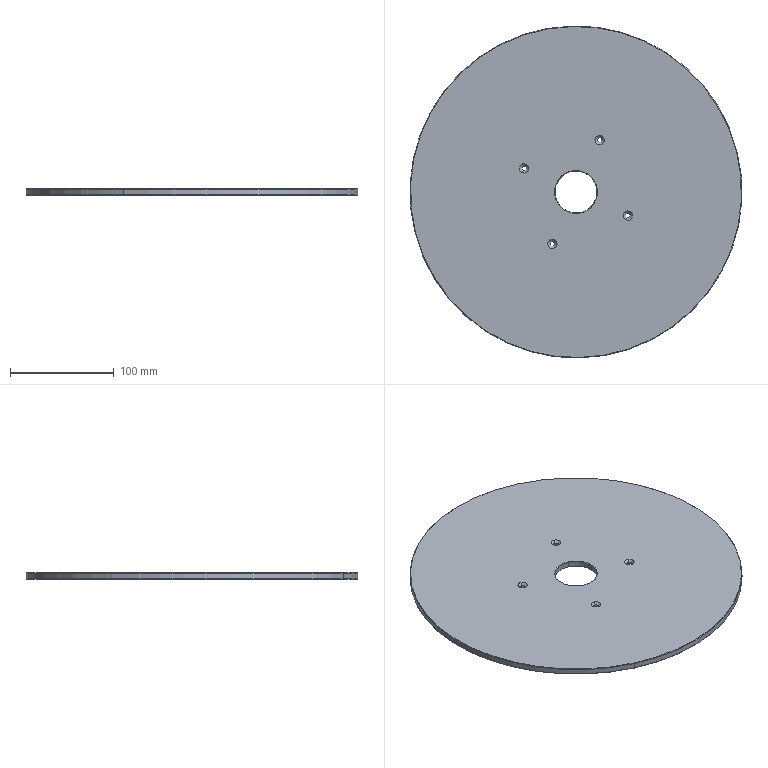Component | SolidWorks | 8TC-A17001-20-04Baffle1-1 | 1 solid | 30 faces | box 320 x 320 x 6 mm | volume 473967 mm3 | cone 16 | cylinder 12 | plane 2 | commonest cylinder face diameters 4.5 x8 40.5 x2 320 x2 | material Tempered Glass
STEP:
#1=COLOUR_RGB('',0.7922,0.8196,0.9333);
#2=FILL_AREA_STYLE_COLOUR('',#1);
#3=FILL_AREA_STYLE('',(#2));
#4=SURFACE_STYLE_FILL_AREA(#3);
#5=SURFACE_SIDE_STYLE('',(#4));
#6=SURFACE_STYLE_USAGE(.BOTH.,#5);
#7=PRESENTATION_STYLE_ASSIGNMENT((#6));
#8=CARTESIAN_POINT('',(26.261,2.186,4.429));
#9=VERTEX_POINT('',#8);
#10=CARTESIAN_POINT('',(31.458,13.619,4.429));
#11=VERTEX_POINT('',#10);
#12=CARTESIAN_POINT('',(28.859,7.902,4.429));
#13=DIRECTION('',(0.,-0.,1.));
#14=DIRECTION('',(-0.4138,-0.9104,0.));
#15=AXIS2_PLACEMENT_3D('',#12,#13,#14);
#16=CIRCLE('',#15,6.28);
#17=EDGE_CURVE('',#9,#11,#16,.T.);
#18=ORIENTED_EDGE('',*,*,#17,.F.);
#19=CARTESIAN_POINT('',(26.253,2.168,4.409));
#20=VERTEX_POINT('',#19);
#21=CARTESIAN_POINT('',(26.261,2.186,4.429));
#22=DIRECTION('',(-0.2926,-0.6437,-0.7071));
#23=VECTOR('',#22,39.37);
#24=LINE('',#21,#23);
#25=EDGE_CURVE('',#9,#20,#24,.T.);
#26=ORIENTED_EDGE('',*,*,#25,.T.);
#27=CARTESIAN_POINT('',(31.466,13.637,4.409));
#28=VERTEX_POINT('',#27);
#29=CARTESIAN_POINT('',(28.859,7.902,4.409));
#30=DIRECTION('',(-0.,0.,-1.));
#31=DIRECTION('',(-0.4138,-0.9104,0.));
#32=AXIS2_PLACEMENT_3D('',#29,#30,#31);
#33=CIRCLE('',#32,6.299);
#34=EDGE_CURVE('',#28,#20,#33,.T.);
#35=ORIENTED_EDGE('',*,*,#34,.F.);
#36=CARTESIAN_POINT('',(31.458,13.619,4.429));
#37=DIRECTION('',(0.2926,0.6437,-0.7071));
#38=VECTOR('',#37,39.37);
#39=LINE('',#36,#38);
#40=EDGE_CURVE('',#11,#28,#39,.T.);
#41=ORIENTED_EDGE('',*,*,#40,.F.);
#42=EDGE_LOOP('',(#18,#26,#35,#41));
#43=FACE_OUTER_BOUND('',#42,.T.);
#44=CARTESIAN_POINT('',(28.859,7.902,4.429));
#45=DIRECTION('',(-0.,0.,-1.));
#46=DIRECTION('',(0.4138,0.9104,0.));
#47=AXIS2_PLACEMENT_3D('',#44,#45,#46);
#48=CONICAL_SURFACE('',#47,6.28,0.7854);
#49=ADVANCED_FACE('',(#43),#48,.T.);
#50=CARTESIAN_POINT('',(31.458,13.619,4.193));
#51=VERTEX_POINT('',#50);
#52=CARTESIAN_POINT('',(26.261,2.186,4.193));
#53=VERTEX_POINT('',#52);
#54=CARTESIAN_POINT('',(28.859,7.902,4.193));
#55=DIRECTION('',(-0.,0.,-1.));
#56=DIRECTION('',(-0.4138,-0.9104,0.));
#57=AXIS2_PLACEMENT_3D('',#54,#55,#56);
#58=CIRCLE('',#57,6.28);
#59=EDGE_CURVE('',#51,#53,#58,.T.);
#60=ORIENTED_EDGE('',*,*,#59,.F.);
#61=CARTESIAN_POINT('',(31.466,13.637,4.213));
#62=VERTEX_POINT('',#61);
#63=CARTESIAN_POINT('',(31.466,13.637,4.213));
#64=DIRECTION('',(0.2926,0.6437,0.7071));
#65=VECTOR('',#64,39.37);
#66=LINE('',#63,#65);
#67=EDGE_CURVE('',#51,#62,#66,.T.);
#68=ORIENTED_EDGE('',*,*,#67,.T.);
#69=CARTESIAN_POINT('',(26.253,2.168,4.213));
#70=VERTEX_POINT('',#69);
#71=CARTESIAN_POINT('',(28.859,7.902,4.213));
#72=DIRECTION('',(0.,-0.,1.));
#73=DIRECTION('',(-0.4138,-0.9104,0.));
#74=AXIS2_PLACEMENT_3D('',#71,#72,#73);
#75=CIRCLE('',#74,6.299);
#76=EDGE_CURVE('',#70,#62,#75,.T.);
#77=ORIENTED_EDGE('',*,*,#76,.F.);
#78=CARTESIAN_POINT('',(26.253,2.168,4.213));
#79=DIRECTION('',(-0.2926,-0.6437,0.7071));
#80=VECTOR('',#79,39.37);
#81=LINE('',#78,#80);
#82=EDGE_CURVE('',#53,#70,#81,.T.);
#83=ORIENTED_EDGE('',*,*,#82,.F.);
#84=EDGE_LOOP('',(#60,#68,#77,#83));
#85=FACE_OUTER_BOUND('',#84,.T.);
#86=CARTESIAN_POINT('',(28.859,7.902,4.213));
#87=DIRECTION('',(0.,-0.,1.));
#88=DIRECTION('',(-0.4138,-0.9104,0.));
#89=AXIS2_PLACEMENT_3D('',#86,#87,#88);
#90=CONICAL_SURFACE('',#89,6.299,0.7854);
#91=ADVANCED_FACE('',(#85),#90,.T.);
#92=CARTESIAN_POINT('',(29.189,8.628,4.409));
#93=VERTEX_POINT('',#92);
#94=CARTESIAN_POINT('',(28.53,7.177,4.409));
#95=VERTEX_POINT('',#94);
#96=CARTESIAN_POINT('',(28.859,7.902,4.409));
#97=DIRECTION('',(0.,-0.,1.));
#98=DIRECTION('',(-0.4138,-0.9104,0.));
#99=AXIS2_PLACEMENT_3D('',#96,#97,#98);
#100=CIRCLE('',#99,0.7972);
#101=EDGE_CURVE('',#93,#95,#100,.T.);
#102=ORIENTED_EDGE('',*,*,#101,.F.);
#103=CARTESIAN_POINT('',(29.197,8.646,4.429));
#104=VERTEX_POINT('',#103);
#105=CARTESIAN_POINT('',(29.189,8.628,4.409));
#106=DIRECTION('',(0.2926,0.6437,0.7071));
#107=VECTOR('',#106,39.37);
#108=LINE('',#105,#107);
#109=EDGE_CURVE('',#93,#104,#108,.T.);
#110=ORIENTED_EDGE('',*,*,#109,.T.);
#111=CARTESIAN_POINT('',(28.521,7.159,4.429));
#112=VERTEX_POINT('',#111);
#113=CARTESIAN_POINT('',(28.859,7.902,4.429));
#114=DIRECTION('',(-0.,0.,-1.));
#115=DIRECTION('',(-0.4138,-0.9104,0.));
#116=AXIS2_PLACEMENT_3D('',#113,#114,#115);
#117=CIRCLE('',#116,0.8169);
#118=EDGE_CURVE('',#112,#104,#117,.T.);
#119=ORIENTED_EDGE('',*,*,#118,.F.);
#120=CARTESIAN_POINT('',(28.53,7.177,4.409));
#121=DIRECTION('',(-0.2926,-0.6437,0.7071));
#122=VECTOR('',#121,39.37);
#123=LINE('',#120,#122);
#124=EDGE_CURVE('',#95,#112,#123,.T.);
#125=ORIENTED_EDGE('',*,*,#124,.F.);
#126=EDGE_LOOP('',(#102,#110,#119,#125));
#127=FACE_OUTER_BOUND('',#126,.T.);
#128=CARTESIAN_POINT('',(28.859,7.902,4.409));
#129=DIRECTION('',(0.,-0.,1.));
#130=DIRECTION('',(-0.4138,-0.9104,0.));
#131=AXIS2_PLACEMENT_3D('',#128,#129,#130);
#132=CONICAL_SURFACE('',#131,0.7972,0.7854);
#133=ADVANCED_FACE('',(#127),#132,.F.);
#134=CARTESIAN_POINT('',(28.53,7.177,4.213));
#135=VERTEX_POINT('',#134);
#136=CARTESIAN_POINT('',(29.189,8.628,4.213));
#137=VERTEX_POINT('',#136);
#138=CARTESIAN_POINT('',(28.859,7.902,4.213));
#139=DIRECTION('',(-0.,0.,-1.));
#140=DIRECTION('',(-0.4138,-0.9104,0.));
#141=AXIS2_PLACEMENT_3D('',#138,#139,#140);
#142=CIRCLE('',#141,0.7972);
#143=EDGE_CURVE('',#135,#137,#142,.T.);
#144=ORIENTED_EDGE('',*,*,#143,.F.);
#145=CARTESIAN_POINT('',(28.521,7.159,4.193));
#146=VERTEX_POINT('',#145);
#147=CARTESIAN_POINT('',(28.521,7.159,4.193));
#148=DIRECTION('',(-0.2926,-0.6437,-0.7071));
#149=VECTOR('',#148,39.37);
#150=LINE('',#147,#149);
#151=EDGE_CURVE('',#135,#146,#150,.T.);
#152=ORIENTED_EDGE('',*,*,#151,.T.);
#153=CARTESIAN_POINT('',(29.197,8.646,4.193));
#154=VERTEX_POINT('',#153);
#155=CARTESIAN_POINT('',(28.859,7.902,4.193));
#156=DIRECTION('',(0.,-0.,1.));
#157=DIRECTION('',(-0.4138,-0.9104,0.));
#158=AXIS2_PLACEMENT_3D('',#155,#156,#157);
#159=CIRCLE('',#158,0.8169);
#160=EDGE_CURVE('',#154,#146,#159,.T.);
#161=ORIENTED_EDGE('',*,*,#160,.F.);
#162=CARTESIAN_POINT('',(29.197,8.646,4.193));
#163=DIRECTION('',(0.2926,0.6437,-0.7071));
#164=VECTOR('',#163,39.37);
#165=LINE('',#162,#164);
#166=EDGE_CURVE('',#137,#154,#165,.T.);
#167=ORIENTED_EDGE('',*,*,#166,.F.);
#168=EDGE_LOOP('',(#144,#152,#161,#167));
#169=FACE_OUTER_BOUND('',#168,.T.);
#170=CARTESIAN_POINT('',(28.859,7.902,4.193));
#171=DIRECTION('',(-0.,0.,-1.));
#172=DIRECTION('',(0.4138,0.9104,0.));
#173=AXIS2_PLACEMENT_3D('',#170,#171,#172);
#174=CONICAL_SURFACE('',#173,0.8169,0.7854);
#175=ADVANCED_FACE('',(#169),#174,.F.);
#176=CARTESIAN_POINT('',(30.867,7.087,4.341));
#177=VERTEX_POINT('',#176);
#178=CARTESIAN_POINT('',(30.794,6.926,4.341));
#179=VERTEX_POINT('',#178);
#180=CARTESIAN_POINT('',(30.831,7.006,4.341));
#181=DIRECTION('',(0.,-0.,1.));
#182=DIRECTION('',(-0.4138,-0.9104,0.));
#183=AXIS2_PLACEMENT_3D('',#180,#181,#182);
#184=CIRCLE('',#183,0.08858);
#185=EDGE_CURVE('',#177,#179,#184,.T.);
#186=ORIENTED_EDGE('',*,*,#185,.F.);
#187=CARTESIAN_POINT('',(30.904,7.167,4.429));
#188=VERTEX_POINT('',#187);
#189=CARTESIAN_POINT('',(30.904,7.167,4.429));
#190=DIRECTION('',(0.2926,0.6437,0.7071));
#191=VECTOR('',#190,39.37);
#192=LINE('',#189,#191);
#193=EDGE_CURVE('',#177,#188,#192,.T.);
#194=ORIENTED_EDGE('',*,*,#193,.T.);
#195=CARTESIAN_POINT('',(30.758,6.846,4.429));
#196=VERTEX_POINT('',#195);
#197=CARTESIAN_POINT('',(30.831,7.006,4.429));
#198=DIRECTION('',(0.,-0.,1.));
#199=DIRECTION('',(-0.4138,-0.9104,0.));
#200=AXIS2_PLACEMENT_3D('',#197,#198,#199);
#201=CIRCLE('',#200,0.1764);
#202=EDGE_CURVE('',#188,#196,#201,.T.);
#203=ORIENTED_EDGE('',*,*,#202,.T.);
#204=CARTESIAN_POINT('',(30.758,6.846,4.429));
#205=DIRECTION('',(-0.2926,-0.6437,0.7071));
#206=VECTOR('',#205,39.37);
#207=LINE('',#204,#206);
#208=EDGE_CURVE('',#179,#196,#207,.T.);
#209=ORIENTED_EDGE('',*,*,#208,.F.);
#210=EDGE_LOOP('',(#186,#194,#203,#209));
#211=FACE_OUTER_BOUND('',#210,.T.);
#212=CARTESIAN_POINT('',(30.831,7.006,4.429));
#213=DIRECTION('',(0.,-0.,1.));
#214=DIRECTION('',(-0.4138,-0.9104,0.));
#215=AXIS2_PLACEMENT_3D('',#212,#213,#214);
#216=CONICAL_SURFACE('',#215,0.1764,0.7854);
#217=ADVANCED_FACE('',(#211),#216,.F.);
#218=CARTESIAN_POINT('',(30.867,7.087,4.193));
#219=VERTEX_POINT('',#218);
#220=CARTESIAN_POINT('',(30.794,6.926,4.193));
#221=VERTEX_POINT('',#220);
#222=CARTESIAN_POINT('',(30.831,7.006,4.193));
#223=DIRECTION('',(0.,-0.,1.));
#224=DIRECTION('',(-0.4138,-0.9104,0.));
#225=AXIS2_PLACEMENT_3D('',#222,#223,#224);
#226=CIRCLE('',#225,0.08858);
#227=EDGE_CURVE('',#219,#221,#226,.T.);
#228=ORIENTED_EDGE('',*,*,#227,.F.);
#229=CARTESIAN_POINT('',(30.867,7.087,4.429));
#230=DIRECTION('',(0.,-0.,1.));
#231=VECTOR('',#230,39.37);
#232=LINE('',#229,#231);
#233=EDGE_CURVE('',#219,#177,#232,.T.);
#234=ORIENTED_EDGE('',*,*,#233,.T.);
#235=ORIENTED_EDGE('',*,*,#185,.T.);
#236=CARTESIAN_POINT('',(30.794,6.926,4.429));
#237=DIRECTION('',(0.,-0.,1.));
#238=VECTOR('',#237,39.37);
#239=LINE('',#236,#238);
#240=EDGE_CURVE('',#221,#179,#239,.T.);
#241=ORIENTED_EDGE('',*,*,#240,.F.);
#242=EDGE_LOOP('',(#228,#234,#235,#241));
#243=FACE_OUTER_BOUND('',#242,.T.);
#244=CARTESIAN_POINT('',(30.831,7.006,4.429));
#245=DIRECTION('',(0.,-0.,1.));
#246=DIRECTION('',(-0.4138,-0.9104,0.));
#247=AXIS2_PLACEMENT_3D('',#244,#245,#246);
#248=CYLINDRICAL_SURFACE('',#247,0.08858);
#249=ADVANCED_FACE('',(#243),#248,.F.);
#250=CARTESIAN_POINT('',(29.792,9.954,4.341));
#251=VERTEX_POINT('',#250);
#252=CARTESIAN_POINT('',(29.719,9.793,4.341));
#253=VERTEX_POINT('',#252);
#254=CARTESIAN_POINT('',(29.755,9.874,4.341));
#255=DIRECTION('',(0.,-0.,1.));
#256=DIRECTION('',(-0.4138,-0.9104,0.));
#257=AXIS2_PLACEMENT_3D('',#254,#255,#256);
#258=CIRCLE('',#257,0.08858);
#259=EDGE_CURVE('',#251,#253,#258,.T.);
#260=ORIENTED_EDGE('',*,*,#259,.F.);
#261=CARTESIAN_POINT('',(29.828,10.034,4.429));
#262=VERTEX_POINT('',#261);
#263=CARTESIAN_POINT('',(29.828,10.034,4.429));
#264=DIRECTION('',(0.2926,0.6437,0.7071));
#265=VECTOR('',#264,39.37);
#266=LINE('',#263,#265);
#267=EDGE_CURVE('',#251,#262,#266,.T.);
#268=ORIENTED_EDGE('',*,*,#267,.T.);
#269=CARTESIAN_POINT('',(29.682,9.713,4.429));
#270=VERTEX_POINT('',#269);
#271=CARTESIAN_POINT('',(29.755,9.874,4.429));
#272=DIRECTION('',(0.,-0.,1.));
#273=DIRECTION('',(-0.4138,-0.9104,0.));
#274=AXIS2_PLACEMENT_3D('',#271,#272,#273);
#275=CIRCLE('',#274,0.1764);
#276=EDGE_CURVE('',#262,#270,#275,.T.);
#277=ORIENTED_EDGE('',*,*,#276,.T.);
#278=CARTESIAN_POINT('',(29.682,9.713,4.429));
#279=DIRECTION('',(-0.2926,-0.6437,0.7071));
#280=VECTOR('',#279,39.37);
#281=LINE('',#278,#280);
#282=EDGE_CURVE('',#253,#270,#281,.T.);
#283=ORIENTED_EDGE('',*,*,#282,.F.);
#284=EDGE_LOOP('',(#260,#268,#277,#283));
#285=FACE_OUTER_BOUND('',#284,.T.);
#286=CARTESIAN_POINT('',(29.755,9.874,4.429));
#287=DIRECTION('',(0.,-0.,1.));
#288=DIRECTION('',(-0.4138,-0.9104,0.));
#289=AXIS2_PLACEMENT_3D('',#286,#287,#288);
#290=CONICAL_SURFACE('',#289,0.1764,0.7854);
#291=ADVANCED_FACE('',(#285),#290,.F.);
#292=CARTESIAN_POINT('',(29.792,9.954,4.193));
#293=VERTEX_POINT('',#292);
#294=CARTESIAN_POINT('',(29.719,9.793,4.193));
#295=VERTEX_POINT('',#294);
#296=CARTESIAN_POINT('',(29.755,9.874,4.193));
#297=DIRECTION('',(0.,-0.,1.));
#298=DIRECTION('',(-0.4138,-0.9104,0.));
#299=AXIS2_PLACEMENT_3D('',#296,#297,#298);
#300=CIRCLE('',#299,0.08858);
#301=EDGE_CURVE('',#293,#295,#300,.T.);
#302=ORIENTED_EDGE('',*,*,#301,.F.);
#303=CARTESIAN_POINT('',(29.792,9.954,4.429));
#304=DIRECTION('',(0.,-0.,1.));
#305=VECTOR('',#304,39.37);
#306=LINE('',#303,#305);
#307=EDGE_CURVE('',#293,#251,#306,.T.);
#308=ORIENTED_EDGE('',*,*,#307,.T.);
#309=ORIENTED_EDGE('',*,*,#259,.T.);
#310=CARTESIAN_POINT('',(29.719,9.793,4.429));
#311=DIRECTION('',(0.,-0.,1.));
#312=VECTOR('',#311,39.37);
#313=LINE('',#310,#312);
#314=EDGE_CURVE('',#295,#253,#313,.T.);
#315=ORIENTED_EDGE('',*,*,#314,.F.);
#316=EDGE_LOOP('',(#302,#308,#309,#315));
#317=FACE_OUTER_BOUND('',#316,.T.);
#318=CARTESIAN_POINT('',(29.755,9.874,4.429));
#319=DIRECTION('',(0.,-0.,1.));
#320=DIRECTION('',(-0.4138,-0.9104,0.));
#321=AXIS2_PLACEMENT_3D('',#318,#319,#320);
#322=CYLINDRICAL_SURFACE('',#321,0.08858);
#323=ADVANCED_FACE('',(#317),#322,.F.);
#324=CARTESIAN_POINT('',(28.,6.012,4.341));
#325=VERTEX_POINT('',#324);
#326=CARTESIAN_POINT('',(27.927,5.851,4.341));
#327=VERTEX_POINT('',#326);
#328=CARTESIAN_POINT('',(27.963,5.931,4.341));
#329=DIRECTION('',(0.,-0.,1.));
#330=DIRECTION('',(-0.4138,-0.9104,0.));
#331=AXIS2_PLACEMENT_3D('',#328,#329,#330);
#332=CIRCLE('',#331,0.08858);
#333=EDGE_CURVE('',#325,#327,#332,.T.);
#334=ORIENTED_EDGE('',*,*,#333,.F.);
#335=CARTESIAN_POINT('',(28.036,6.092,4.429));
#336=VERTEX_POINT('',#335);
#337=CARTESIAN_POINT('',(28.036,6.092,4.429));
#338=DIRECTION('',(0.2926,0.6437,0.7071));
#339=VECTOR('',#338,39.37);
#340=LINE('',#337,#339);
#341=EDGE_CURVE('',#325,#336,#340,.T.);
#342=ORIENTED_EDGE('',*,*,#341,.T.);
#343=CARTESIAN_POINT('',(27.89,5.771,4.429));
#344=VERTEX_POINT('',#343);
#345=CARTESIAN_POINT('',(27.963,5.931,4.429));
#346=DIRECTION('',(0.,-0.,1.));
#347=DIRECTION('',(-0.4138,-0.9104,0.));
#348=AXIS2_PLACEMENT_3D('',#345,#346,#347);
#349=CIRCLE('',#348,0.1764);
#350=EDGE_CURVE('',#336,#344,#349,.T.);
#351=ORIENTED_EDGE('',*,*,#350,.T.);
#352=CARTESIAN_POINT('',(27.89,5.771,4.429));
#353=DIRECTION('',(-0.2926,-0.6437,0.7071));
#354=VECTOR('',#353,39.37);
#355=LINE('',#352,#354);
#356=EDGE_CURVE('',#327,#344,#355,.T.);
#357=ORIENTED_EDGE('',*,*,#356,.F.);
#358=EDGE_LOOP('',(#334,#342,#351,#357));
#359=FACE_OUTER_BOUND('',#358,.T.);
#360=CARTESIAN_POINT('',(27.963,5.931,4.429));
#361=DIRECTION('',(0.,-0.,1.));
#362=DIRECTION('',(-0.4138,-0.9104,0.));
#363=AXIS2_PLACEMENT_3D('',#360,#361,#362);
#364=CONICAL_SURFACE('',#363,0.1764,0.7854);
#365=ADVANCED_FACE('',(#359),#364,.F.);
#366=CARTESIAN_POINT('',(28.,6.012,4.193));
#367=VERTEX_POINT('',#366);
#368=CARTESIAN_POINT('',(27.927,5.851,4.193));
#369=VERTEX_POINT('',#368);
#370=CARTESIAN_POINT('',(27.963,5.931,4.193));
#371=DIRECTION('',(0.,-0.,1.));
#372=DIRECTION('',(-0.4138,-0.9104,0.));
#373=AXIS2_PLACEMENT_3D('',#370,#371,#372);
#374=CIRCLE('',#373,0.08858);
#375=EDGE_CURVE('',#367,#369,#374,.T.);
#376=ORIENTED_EDGE('',*,*,#375,.F.);
#377=CARTESIAN_POINT('',(28.,6.012,4.429));
#378=DIRECTION('',(0.,-0.,1.));
#379=VECTOR('',#378,39.37);
#380=LINE('',#377,#379);
#381=EDGE_CURVE('',#367,#325,#380,.T.);
#382=ORIENTED_EDGE('',*,*,#381,.T.);
#383=ORIENTED_EDGE('',*,*,#333,.T.);
#384=CARTESIAN_POINT('',(27.927,5.851,4.429));
#385=DIRECTION('',(0.,-0.,1.));
#386=VECTOR('',#385,39.37);
#387=LINE('',#384,#386);
#388=EDGE_CURVE('',#369,#327,#387,.T.);
#389=ORIENTED_EDGE('',*,*,#388,.F.);
#390=EDGE_LOOP('',(#376,#382,#383,#389));
#391=FACE_OUTER_BOUND('',#390,.T.);
#392=CARTESIAN_POINT('',(27.963,5.931,4.429));
#393=DIRECTION('',(0.,-0.,1.));
#394=DIRECTION('',(-0.4138,-0.9104,0.));
#395=AXIS2_PLACEMENT_3D('',#392,#393,#394);
#396=CYLINDRICAL_SURFACE('',#395,0.08858);
#397=ADVANCED_FACE('',(#391),#396,.F.);
#398=CARTESIAN_POINT('',(26.925,8.879,4.341));
#399=VERTEX_POINT('',#398);
#400=CARTESIAN_POINT('',(26.851,8.718,4.341));
#401=VERTEX_POINT('',#400);
#402=CARTESIAN_POINT('',(26.888,8.798,4.341));
#403=DIRECTION('',(0.,-0.,1.));
#404=DIRECTION('',(-0.4138,-0.9104,0.));
#405=AXIS2_PLACEMENT_3D('',#402,#403,#404);
#406=CIRCLE('',#405,0.08858);
#407=EDGE_CURVE('',#399,#401,#406,.T.);
#408=ORIENTED_EDGE('',*,*,#407,.F.);
#409=CARTESIAN_POINT('',(26.961,8.959,4.429));
#410=VERTEX_POINT('',#409);
#411=CARTESIAN_POINT('',(26.961,8.959,4.429));
#412=DIRECTION('',(0.2926,0.6437,0.7071));
#413=VECTOR('',#412,39.37);
#414=LINE('',#411,#413);
#415=EDGE_CURVE('',#399,#410,#414,.T.);
#416=ORIENTED_EDGE('',*,*,#415,.T.);
#417=CARTESIAN_POINT('',(26.815,8.638,4.429));
#418=VERTEX_POINT('',#417);
#419=CARTESIAN_POINT('',(26.888,8.798,4.429));
#420=DIRECTION('',(0.,-0.,1.));
#421=DIRECTION('',(-0.4138,-0.9104,0.));
#422=AXIS2_PLACEMENT_3D('',#419,#420,#421);
#423=CIRCLE('',#422,0.1764);
#424=EDGE_CURVE('',#410,#418,#423,.T.);
#425=ORIENTED_EDGE('',*,*,#424,.T.);
#426=CARTESIAN_POINT('',(26.815,8.638,4.429));
#427=DIRECTION('',(-0.2926,-0.6437,0.7071));
#428=VECTOR('',#427,39.37);
#429=LINE('',#426,#428);
#430=EDGE_CURVE('',#401,#418,#429,.T.);
#431=ORIENTED_EDGE('',*,*,#430,.F.);
#432=EDGE_LOOP('',(#408,#416,#425,#431));
#433=FACE_OUTER_BOUND('',#432,.T.);
#434=CARTESIAN_POINT('',(26.888,8.798,4.429));
#435=DIRECTION('',(0.,-0.,1.));
#436=DIRECTION('',(-0.4138,-0.9104,0.));
#437=AXIS2_PLACEMENT_3D('',#434,#435,#436);
#438=CONICAL_SURFACE('',#437,0.1764,0.7854);
#439=ADVANCED_FACE('',(#433),#438,.F.);
#440=CARTESIAN_POINT('',(26.925,8.879,4.193));
#441=VERTEX_POINT('',#440);
#442=CARTESIAN_POINT('',(26.851,8.718,4.193));
#443=VERTEX_POINT('',#442);
#444=CARTESIAN_POINT('',(26.888,8.798,4.193));
#445=DIRECTION('',(0.,-0.,1.));
#446=DIRECTION('',(-0.4138,-0.9104,0.));
#447=AXIS2_PLACEMENT_3D('',#444,#445,#446);
#448=CIRCLE('',#447,0.08858);
#449=EDGE_CURVE('',#441,#443,#448,.T.);
#450=ORIENTED_EDGE('',*,*,#449,.F.);
#451=CARTESIAN_POINT('',(26.925,8.879,4.429));
#452=DIRECTION('',(0.,-0.,1.));
#453=VECTOR('',#452,39.37);
#454=LINE('',#451,#453);
#455=EDGE_CURVE('',#441,#399,#454,.T.);
#456=ORIENTED_EDGE('',*,*,#455,.T.);
#457=ORIENTED_EDGE('',*,*,#407,.T.);
#458=CARTESIAN_POINT('',(26.851,8.718,4.429));
#459=DIRECTION('',(0.,-0.,1.));
#460=VECTOR('',#459,39.37);
#461=LINE('',#458,#460);
#462=EDGE_CURVE('',#443,#401,#461,.T.);
#463=ORIENTED_EDGE('',*,*,#462,.F.);
#464=EDGE_LOOP('',(#450,#456,#457,#463));
#465=FACE_OUTER_BOUND('',#464,.T.);
#466=CARTESIAN_POINT('',(26.888,8.798,4.429));
#467=DIRECTION('',(0.,-0.,1.));
#468=DIRECTION('',(-0.4138,-0.9104,0.));
#469=AXIS2_PLACEMENT_3D('',#466,#467,#468);
#470=CYLINDRICAL_SURFACE('',#469,0.08858);
#471=ADVANCED_FACE('',(#465),#470,.F.);
#472=ORIENTED_EDGE('',*,*,#101,.T.);
#473=CARTESIAN_POINT('',(28.53,7.177,4.429));
#474=DIRECTION('',(-0.,0.,-1.));
#475=VECTOR('',#474,39.37);
#476=LINE('',#473,#475);
#477=EDGE_CURVE('',#95,#135,#476,.T.);
#478=ORIENTED_EDGE('',*,*,#477,.T.);
#479=ORIENTED_EDGE('',*,*,#143,.T.);
#480=CARTESIAN_POINT('',(29.189,8.628,4.429));
#481=DIRECTION('',(-0.,0.,-1.));
#482=VECTOR('',#481,39.37);
#483=LINE('',#480,#482);
#484=EDGE_CURVE('',#93,#137,#483,.T.);
#485=ORIENTED_EDGE('',*,*,#484,.F.);
#486=EDGE_LOOP('',(#472,#478,#479,#485));
#487=FACE_OUTER_BOUND('',#486,.T.);
#488=CARTESIAN_POINT('',(28.859,7.902,4.429));
#489=DIRECTION('',(-0.,0.,-1.));
#490=DIRECTION('',(0.4138,0.9104,0.));
#491=AXIS2_PLACEMENT_3D('',#488,#489,#490);
#492=CYLINDRICAL_SURFACE('',#491,0.7972);
#493=ADVANCED_FACE('',(#487),#492,.F.);
#494=ORIENTED_EDGE('',*,*,#34,.T.);
#495=CARTESIAN_POINT('',(26.253,2.168,4.429));
#496=DIRECTION('',(-0.,0.,-1.));
#497=VECTOR('',#496,39.37);
#498=LINE('',#495,#497);
#499=EDGE_CURVE('',#20,#70,#498,.T.);
#500=ORIENTED_EDGE('',*,*,#499,.T.);
#501=ORIENTED_EDGE('',*,*,#76,.T.);
#502=CARTESIAN_POINT('',(31.466,13.637,4.429));
#503=DIRECTION('',(-0.,0.,-1.));
#504=VECTOR('',#503,39.37);
#505=LINE('',#502,#504);
#506=EDGE_CURVE('',#28,#62,#505,.T.);
#507=ORIENTED_EDGE('',*,*,#506,.F.);
#508=EDGE_LOOP('',(#494,#500,#501,#507));
#509=FACE_OUTER_BOUND('',#508,.T.);
#510=CARTESIAN_POINT('',(28.859,7.902,4.429));
#511=DIRECTION('',(-0.,0.,-1.));
#512=DIRECTION('',(0.4138,0.9104,0.));
#513=AXIS2_PLACEMENT_3D('',#510,#511,#512);
#514=CYLINDRICAL_SURFACE('',#513,6.299);
#515=ADVANCED_FACE('',(#509),#514,.T.);
#516=ORIENTED_EDGE('',*,*,#118,.T.);
#517=CARTESIAN_POINT('',(28.859,7.902,4.429));
#518=DIRECTION('',(-0.,0.,-1.));
#519=DIRECTION('',(-0.4138,-0.9104,0.));
#520=AXIS2_PLACEMENT_3D('',#517,#518,#519);
#521=CIRCLE('',#520,0.8169);
#522=EDGE_CURVE('',#104,#112,#521,.T.);
#523=ORIENTED_EDGE('',*,*,#522,.T.);
#524=EDGE_LOOP('',(#516,#523));
#525=FACE_BOUND('',#524,.T.);
#526=CARTESIAN_POINT('',(28.859,7.902,4.429));
#527=DIRECTION('',(0.,-0.,1.));
#528=DIRECTION('',(-0.4138,-0.9104,0.));
#529=AXIS2_PLACEMENT_3D('',#526,#527,#528);
#530=CIRCLE('',#529,6.28);
#531=EDGE_CURVE('',#11,#9,#530,.T.);
#532=ORIENTED_EDGE('',*,*,#531,.T.);
#533=ORIENTED_EDGE('',*,*,#17,.T.);
#534=EDGE_LOOP('',(#532,#533));
#535=FACE_OUTER_BOUND('',#534,.T.);
#536=CARTESIAN_POINT('',(30.831,7.006,4.429));
#537=DIRECTION('',(0.,-0.,1.));
#538=DIRECTION('',(-0.4138,-0.9104,0.));
#539=AXIS2_PLACEMENT_3D('',#536,#537,#538);
#540=CIRCLE('',#539,0.1764);
#541=EDGE_CURVE('',#196,#188,#540,.T.);
#542=ORIENTED_EDGE('',*,*,#541,.F.);
#543=ORIENTED_EDGE('',*,*,#202,.F.);
#544=EDGE_LOOP('',(#542,#543));
#545=FACE_BOUND('',#544,.T.);
#546=CARTESIAN_POINT('',(29.755,9.874,4.429));
#547=DIRECTION('',(0.,-0.,1.));
#548=DIRECTION('',(-0.4138,-0.9104,0.));
#549=AXIS2_PLACEMENT_3D('',#546,#547,#548);
#550=CIRCLE('',#549,0.1764);
#551=EDGE_CURVE('',#270,#262,#550,.T.);
#552=ORIENTED_EDGE('',*,*,#551,.F.);
#553=ORIENTED_EDGE('',*,*,#276,.F.);
#554=EDGE_LOOP('',(#552,#553));
#555=FACE_BOUND('',#554,.T.);
#556=CARTESIAN_POINT('',(27.963,5.931,4.429));
#557=DIRECTION('',(0.,-0.,1.));
#558=DIRECTION('',(-0.4138,-0.9104,0.));
#559=AXIS2_PLACEMENT_3D('',#556,#557,#558);
#560=CIRCLE('',#559,0.1764);
#561=EDGE_CURVE('',#344,#336,#560,.T.);
#562=ORIENTED_EDGE('',*,*,#561,.F.);
#563=ORIENTED_EDGE('',*,*,#350,.F.);
#564=EDGE_LOOP('',(#562,#563));
#565=FACE_BOUND('',#564,.T.);
#566=CARTESIAN_POINT('',(26.888,8.798,4.429));
#567=DIRECTION('',(0.,-0.,1.));
#568=DIRECTION('',(-0.4138,-0.9104,0.));
#569=AXIS2_PLACEMENT_3D('',#566,#567,#568);
#570=CIRCLE('',#569,0.1764);
#571=EDGE_CURVE('',#418,#410,#570,.T.);
#572=ORIENTED_EDGE('',*,*,#571,.F.);
#573=ORIENTED_EDGE('',*,*,#424,.F.);
#574=EDGE_LOOP('',(#572,#573));
#575=FACE_BOUND('',#574,.T.);
#576=CARTESIAN_POINT('',(28.859,7.902,4.429));
#577=DIRECTION('',(0.,-0.,1.));
#578=DIRECTION('',(-0.4138,-0.9104,0.));
#579=AXIS2_PLACEMENT_3D('',#576,#577,#578);
#580=PLANE('',#579);
#581=ADVANCED_FACE('',(#525,#535,#545,#555,#565,#575),#580,.T.);
#582=ORIENTED_EDGE('',*,*,#160,.T.);
#583=CARTESIAN_POINT('',(28.859,7.902,4.193));
#584=DIRECTION('',(0.,-0.,1.));
#585=DIRECTION('',(-0.4138,-0.9104,0.));
#586=AXIS2_PLACEMENT_3D('',#583,#584,#585);
#587=CIRCLE('',#586,0.8169);
#588=EDGE_CURVE('',#146,#154,#587,.T.);
#589=ORIENTED_EDGE('',*,*,#588,.T.);
#590=EDGE_LOOP('',(#582,#589));
#591=FACE_BOUND('',#590,.T.);
#592=CARTESIAN_POINT('',(28.859,7.902,4.193));
#593=DIRECTION('',(-0.,0.,-1.));
#594=DIRECTION('',(-0.4138,-0.9104,0.));
#595=AXIS2_PLACEMENT_3D('',#592,#593,#594);
#596=CIRCLE('',#595,6.28);
#597=EDGE_CURVE('',#53,#51,#596,.T.);
#598=ORIENTED_EDGE('',*,*,#597,.T.);
#599=ORIENTED_EDGE('',*,*,#59,.T.);
#600=EDGE_LOOP('',(#598,#599));
#601=FACE_OUTER_BOUND('',#600,.T.);
#602=CARTESIAN_POINT('',(30.831,7.006,4.193));
#603=DIRECTION('',(0.,-0.,1.));
#604=DIRECTION('',(-0.4138,-0.9104,0.));
#605=AXIS2_PLACEMENT_3D('',#602,#603,#604);
#606=CIRCLE('',#605,0.08858);
#607=EDGE_CURVE('',#221,#219,#606,.T.);
#608=ORIENTED_EDGE('',*,*,#607,.T.);
#609=ORIENTED_EDGE('',*,*,#227,.T.);
#610=EDGE_LOOP('',(#608,#609));
#611=FACE_BOUND('',#610,.T.);
#612=CARTESIAN_POINT('',(29.755,9.874,4.193));
#613=DIRECTION('',(0.,-0.,1.));
#614=DIRECTION('',(-0.4138,-0.9104,0.));
#615=AXIS2_PLACEMENT_3D('',#612,#613,#614);
#616=CIRCLE('',#615,0.08858);
#617=EDGE_CURVE('',#295,#293,#616,.T.);
#618=ORIENTED_EDGE('',*,*,#617,.T.);
#619=ORIENTED_EDGE('',*,*,#301,.T.);
#620=EDGE_LOOP('',(#618,#619));
#621=FACE_BOUND('',#620,.T.);
#622=CARTESIAN_POINT('',(27.963,5.931,4.193));
#623=DIRECTION('',(0.,-0.,1.));
#624=DIRECTION('',(-0.4138,-0.9104,0.));
#625=AXIS2_PLACEMENT_3D('',#622,#623,#624);
#626=CIRCLE('',#625,0.08858);
#627=EDGE_CURVE('',#369,#367,#626,.T.);
#628=ORIENTED_EDGE('',*,*,#627,.T.);
#629=ORIENTED_EDGE('',*,*,#375,.T.);
#630=EDGE_LOOP('',(#628,#629));
#631=FACE_BOUND('',#630,.T.);
#632=CARTESIAN_POINT('',(26.888,8.798,4.193));
#633=DIRECTION('',(0.,-0.,1.));
#634=DIRECTION('',(-0.4138,-0.9104,0.));
#635=AXIS2_PLACEMENT_3D('',#632,#633,#634);
#636=CIRCLE('',#635,0.08858);
#637=EDGE_CURVE('',#443,#441,#636,.T.);
#638=ORIENTED_EDGE('',*,*,#637,.T.);
#639=ORIENTED_EDGE('',*,*,#449,.T.);
#640=EDGE_LOOP('',(#638,#639));
#641=FACE_BOUND('',#640,.T.);
#642=CARTESIAN_POINT('',(28.859,7.902,4.193));
#643=DIRECTION('',(0.,-0.,1.));
#644=DIRECTION('',(-0.4138,-0.9104,0.));
#645=AXIS2_PLACEMENT_3D('',#642,#643,#644);
#646=PLANE('',#645);
#647=ADVANCED_FACE('',(#591,#601,#611,#621,#631,#641),#646,.F.);
#648=ORIENTED_EDGE('',*,*,#499,.F.);
#649=CARTESIAN_POINT('',(28.859,7.902,4.409));
#650=DIRECTION('',(-0.,0.,-1.));
#651=DIRECTION('',(-0.4138,-0.9104,0.));
#652=AXIS2_PLACEMENT_3D('',#649,#650,#651);
#653=CIRCLE('',#652,6.299);
#654=EDGE_CURVE('',#20,#28,#653,.T.);
#655=ORIENTED_EDGE('',*,*,#654,.T.);
#656=ORIENTED_EDGE('',*,*,#506,.T.);
#657=CARTESIAN_POINT('',(28.859,7.902,4.213));
#658=DIRECTION('',(0.,-0.,1.));
#659=DIRECTION('',(-0.4138,-0.9104,0.));
#660=AXIS2_PLACEMENT_3D('',#657,#658,#659);
#661=CIRCLE('',#660,6.299);
#662=EDGE_CURVE('',#62,#70,#661,.T.);
#663=ORIENTED_EDGE('',*,*,#662,.T.);
#664=EDGE_LOOP('',(#648,#655,#656,#663));
#665=FACE_OUTER_BOUND('',#664,.T.);
#666=CARTESIAN_POINT('',(28.859,7.902,4.429));
#667=DIRECTION('',(-0.,0.,-1.));
#668=DIRECTION('',(0.4138,0.9104,0.));
#669=AXIS2_PLACEMENT_3D('',#666,#667,#668);
#670=CYLINDRICAL_SURFACE('',#669,6.299);
#671=ADVANCED_FACE('',(#665),#670,.T.);
#672=ORIENTED_EDGE('',*,*,#477,.F.);
#673=CARTESIAN_POINT('',(28.859,7.902,4.409));
#674=DIRECTION('',(0.,-0.,1.));
#675=DIRECTION('',(-0.4138,-0.9104,0.));
#676=AXIS2_PLACEMENT_3D('',#673,#674,#675);
#677=CIRCLE('',#676,0.7972);
#678=EDGE_CURVE('',#95,#93,#677,.T.);
#679=ORIENTED_EDGE('',*,*,#678,.T.);
#680=ORIENTED_EDGE('',*,*,#484,.T.);
#681=CARTESIAN_POINT('',(28.859,7.902,4.213));
#682=DIRECTION('',(-0.,0.,-1.));
#683=DIRECTION('',(-0.4138,-0.9104,0.));
#684=AXIS2_PLACEMENT_3D('',#681,#682,#683);
#685=CIRCLE('',#684,0.7972);
#686=EDGE_CURVE('',#137,#135,#685,.T.);
#687=ORIENTED_EDGE('',*,*,#686,.T.);
#688=EDGE_LOOP('',(#672,#679,#680,#687));
#689=FACE_OUTER_BOUND('',#688,.T.);
#690=CARTESIAN_POINT('',(28.859,7.902,4.429));
#691=DIRECTION('',(-0.,0.,-1.));
#692=DIRECTION('',(0.4138,0.9104,0.));
#693=AXIS2_PLACEMENT_3D('',#690,#691,#692);
#694=CYLINDRICAL_SURFACE('',#693,0.7972);
#695=ADVANCED_FACE('',(#689),#694,.F.);
#696=ORIENTED_EDGE('',*,*,#455,.F.);
#697=ORIENTED_EDGE('',*,*,#637,.F.);
#698=ORIENTED_EDGE('',*,*,#462,.T.);
#699=CARTESIAN_POINT('',(26.888,8.798,4.341));
#700=DIRECTION('',(0.,-0.,1.));
#701=DIRECTION('',(-0.4138,-0.9104,0.));
#702=AXIS2_PLACEMENT_3D('',#699,#700,#701);
#703=CIRCLE('',#702,0.08858);
#704=EDGE_CURVE('',#401,#399,#703,.T.);
#705=ORIENTED_EDGE('',*,*,#704,.T.);
#706=EDGE_LOOP('',(#696,#697,#698,#705));
#707=FACE_OUTER_BOUND('',#706,.T.);
#708=CARTESIAN_POINT('',(26.888,8.798,4.429));
#709=DIRECTION('',(0.,-0.,1.));
#710=DIRECTION('',(-0.4138,-0.9104,0.));
#711=AXIS2_PLACEMENT_3D('',#708,#709,#710);
#712=CYLINDRICAL_SURFACE('',#711,0.08858);
#713=ADVANCED_FACE('',(#707),#712,.F.);
#714=ORIENTED_EDGE('',*,*,#415,.F.);
#715=ORIENTED_EDGE('',*,*,#704,.F.);
#716=ORIENTED_EDGE('',*,*,#430,.T.);
#717=ORIENTED_EDGE('',*,*,#571,.T.);
#718=EDGE_LOOP('',(#714,#715,#716,#717));
#719=FACE_OUTER_BOUND('',#718,.T.);
#720=CARTESIAN_POINT('',(26.888,8.798,4.429));
#721=DIRECTION('',(0.,-0.,1.));
#722=DIRECTION('',(-0.4138,-0.9104,0.));
#723=AXIS2_PLACEMENT_3D('',#720,#721,#722);
#724=CONICAL_SURFACE('',#723,0.1764,0.7854);
#725=ADVANCED_FACE('',(#719),#724,.F.);
#726=ORIENTED_EDGE('',*,*,#381,.F.);
#727=ORIENTED_EDGE('',*,*,#627,.F.);
#728=ORIENTED_EDGE('',*,*,#388,.T.);
#729=CARTESIAN_POINT('',(27.963,5.931,4.341));
#730=DIRECTION('',(0.,-0.,1.));
#731=DIRECTION('',(-0.4138,-0.9104,0.));
#732=AXIS2_PLACEMENT_3D('',#729,#730,#731);
#733=CIRCLE('',#732,0.08858);
#734=EDGE_CURVE('',#327,#325,#733,.T.);
#735=ORIENTED_EDGE('',*,*,#734,.T.);
#736=EDGE_LOOP('',(#726,#727,#728,#735));
#737=FACE_OUTER_BOUND('',#736,.T.);
#738=CARTESIAN_POINT('',(27.963,5.931,4.429));
#739=DIRECTION('',(0.,-0.,1.));
#740=DIRECTION('',(-0.4138,-0.9104,0.));
#741=AXIS2_PLACEMENT_3D('',#738,#739,#740);
#742=CYLINDRICAL_SURFACE('',#741,0.08858);
#743=ADVANCED_FACE('',(#737),#742,.F.);
#744=ORIENTED_EDGE('',*,*,#341,.F.);
#745=ORIENTED_EDGE('',*,*,#734,.F.);
#746=ORIENTED_EDGE('',*,*,#356,.T.);
#747=ORIENTED_EDGE('',*,*,#561,.T.);
#748=EDGE_LOOP('',(#744,#745,#746,#747));
#749=FACE_OUTER_BOUND('',#748,.T.);
#750=CARTESIAN_POINT('',(27.963,5.931,4.429));
#751=DIRECTION('',(0.,-0.,1.));
#752=DIRECTION('',(-0.4138,-0.9104,0.));
#753=AXIS2_PLACEMENT_3D('',#750,#751,#752);
#754=CONICAL_SURFACE('',#753,0.1764,0.7854);
#755=ADVANCED_FACE('',(#749),#754,.F.);
#756=ORIENTED_EDGE('',*,*,#307,.F.);
#757=ORIENTED_EDGE('',*,*,#617,.F.);
#758=ORIENTED_EDGE('',*,*,#314,.T.);
#759=CARTESIAN_POINT('',(29.755,9.874,4.341));
#760=DIRECTION('',(0.,-0.,1.));
#761=DIRECTION('',(-0.4138,-0.9104,0.));
#762=AXIS2_PLACEMENT_3D('',#759,#760,#761);
#763=CIRCLE('',#762,0.08858);
#764=EDGE_CURVE('',#253,#251,#763,.T.);
#765=ORIENTED_EDGE('',*,*,#764,.T.);
#766=EDGE_LOOP('',(#756,#757,#758,#765));
#767=FACE_OUTER_BOUND('',#766,.T.);
#768=CARTESIAN_POINT('',(29.755,9.874,4.429));
#769=DIRECTION('',(0.,-0.,1.));
#770=DIRECTION('',(-0.4138,-0.9104,0.));
#771=AXIS2_PLACEMENT_3D('',#768,#769,#770);
#772=CYLINDRICAL_SURFACE('',#771,0.08858);
#773=ADVANCED_FACE('',(#767),#772,.F.);
#774=ORIENTED_EDGE('',*,*,#267,.F.);
#775=ORIENTED_EDGE('',*,*,#764,.F.);
#776=ORIENTED_EDGE('',*,*,#282,.T.);
#777=ORIENTED_EDGE('',*,*,#551,.T.);
#778=EDGE_LOOP('',(#774,#775,#776,#777));
#779=FACE_OUTER_BOUND('',#778,.T.);
#780=CARTESIAN_POINT('',(29.755,9.874,4.429));
#781=DIRECTION('',(0.,-0.,1.));
#782=DIRECTION('',(-0.4138,-0.9104,0.));
#783=AXIS2_PLACEMENT_3D('',#780,#781,#782);
#784=CONICAL_SURFACE('',#783,0.1764,0.7854);
#785=ADVANCED_FACE('',(#779),#784,.F.);
#786=ORIENTED_EDGE('',*,*,#233,.F.);
#787=ORIENTED_EDGE('',*,*,#607,.F.);
#788=ORIENTED_EDGE('',*,*,#240,.T.);
#789=CARTESIAN_POINT('',(30.831,7.006,4.341));
#790=DIRECTION('',(0.,-0.,1.));
#791=DIRECTION('',(-0.4138,-0.9104,0.));
#792=AXIS2_PLACEMENT_3D('',#789,#790,#791);
#793=CIRCLE('',#792,0.08858);
#794=EDGE_CURVE('',#179,#177,#793,.T.);
#795=ORIENTED_EDGE('',*,*,#794,.T.);
#796=EDGE_LOOP('',(#786,#787,#788,#795));
#797=FACE_OUTER_BOUND('',#796,.T.);
#798=CARTESIAN_POINT('',(30.831,7.006,4.429));
#799=DIRECTION('',(0.,-0.,1.));
#800=DIRECTION('',(-0.4138,-0.9104,0.));
#801=AXIS2_PLACEMENT_3D('',#798,#799,#800);
#802=CYLINDRICAL_SURFACE('',#801,0.08858);
#803=ADVANCED_FACE('',(#797),#802,.F.);
#804=ORIENTED_EDGE('',*,*,#193,.F.);
#805=ORIENTED_EDGE('',*,*,#794,.F.);
#806=ORIENTED_EDGE('',*,*,#208,.T.);
#807=ORIENTED_EDGE('',*,*,#541,.T.);
#808=EDGE_LOOP('',(#804,#805,#806,#807));
#809=FACE_OUTER_BOUND('',#808,.T.);
#810=CARTESIAN_POINT('',(30.831,7.006,4.429));
#811=DIRECTION('',(0.,-0.,1.));
#812=DIRECTION('',(-0.4138,-0.9104,0.));
#813=AXIS2_PLACEMENT_3D('',#810,#811,#812);
#814=CONICAL_SURFACE('',#813,0.1764,0.7854);
#815=ADVANCED_FACE('',(#809),#814,.F.);
#816=ORIENTED_EDGE('',*,*,#151,.F.);
#817=ORIENTED_EDGE('',*,*,#686,.F.);
#818=ORIENTED_EDGE('',*,*,#166,.T.);
#819=ORIENTED_EDGE('',*,*,#588,.F.);
#820=EDGE_LOOP('',(#816,#817,#818,#819));
#821=FACE_OUTER_BOUND('',#820,.T.);
#822=CARTESIAN_POINT('',(28.859,7.902,4.193));
#823=DIRECTION('',(-0.,0.,-1.));
#824=DIRECTION('',(0.4138,0.9104,0.));
#825=AXIS2_PLACEMENT_3D('',#822,#823,#824);
#826=CONICAL_SURFACE('',#825,0.8169,0.7854);
#827=ADVANCED_FACE('',(#821),#826,.F.);
#828=ORIENTED_EDGE('',*,*,#109,.F.);
#829=ORIENTED_EDGE('',*,*,#678,.F.);
#830=ORIENTED_EDGE('',*,*,#124,.T.);
#831=ORIENTED_EDGE('',*,*,#522,.F.);
#832=EDGE_LOOP('',(#828,#829,#830,#831));
#833=FACE_OUTER_BOUND('',#832,.T.);
#834=CARTESIAN_POINT('',(28.859,7.902,4.409));
#835=DIRECTION('',(0.,-0.,1.));
#836=DIRECTION('',(-0.4138,-0.9104,0.));
#837=AXIS2_PLACEMENT_3D('',#834,#835,#836);
#838=CONICAL_SURFACE('',#837,0.7972,0.7854);
#839=ADVANCED_FACE('',(#833),#838,.F.);
#840=ORIENTED_EDGE('',*,*,#67,.F.);
#841=ORIENTED_EDGE('',*,*,#597,.F.);
#842=ORIENTED_EDGE('',*,*,#82,.T.);
#843=ORIENTED_EDGE('',*,*,#662,.F.);
#844=EDGE_LOOP('',(#840,#841,#842,#843));
#845=FACE_OUTER_BOUND('',#844,.T.);
#846=CARTESIAN_POINT('',(28.859,7.902,4.213));
#847=DIRECTION('',(0.,-0.,1.));
#848=DIRECTION('',(-0.4138,-0.9104,0.));
#849=AXIS2_PLACEMENT_3D('',#846,#847,#848);
#850=CONICAL_SURFACE('',#849,6.299,0.7854);
#851=ADVANCED_FACE('',(#845),#850,.T.);
#852=ORIENTED_EDGE('',*,*,#25,.F.);
#853=ORIENTED_EDGE('',*,*,#531,.F.);
#854=ORIENTED_EDGE('',*,*,#40,.T.);
#855=ORIENTED_EDGE('',*,*,#654,.F.);
#856=EDGE_LOOP('',(#852,#853,#854,#855));
#857=FACE_OUTER_BOUND('',#856,.T.);
#858=CARTESIAN_POINT('',(28.859,7.902,4.429));
#859=DIRECTION('',(-0.,0.,-1.));
#860=DIRECTION('',(0.4138,0.9104,0.));
#861=AXIS2_PLACEMENT_3D('',#858,#859,#860);
#862=CONICAL_SURFACE('',#861,6.28,0.7854);
#863=ADVANCED_FACE('',(#857),#862,.T.);
#864=CLOSED_SHELL('',(#49,#91,#133,#175,#217,#249,#291,#323,#365,#397,#439,#471,#493,#515,#581,#647,#671,#695,#713,#725,#743,#755,#773,#785,#803,#815,#827,#839,#851,#863));
#865=MANIFOLD_SOLID_BREP('',#864);
#866=STYLED_ITEM('',(#7),#865);
#867=PRESENTATION_LAYER_ASSIGNMENT('','',(#866));
#868=(LENGTH_UNIT()NAMED_UNIT(*)SI_UNIT($,.METRE.));
#869=LENGTH_MEASURE_WITH_UNIT(LENGTH_MEASURE(0.0254),#868);
#870=DIMENSIONAL_EXPONENTS(1.,0.,0.,0.,0.,0.,0.);
#871=(CONVERSION_BASED_UNIT('',#869)LENGTH_UNIT()NAMED_UNIT(#870));
#872=UNCERTAINTY_MEASURE_WITH_UNIT(LENGTH_MEASURE(0.00001),#871,'','');
#873=(NAMED_UNIT(*)PLANE_ANGLE_UNIT()SI_UNIT($,.RADIAN.));
#874=(NAMED_UNIT(*)SI_UNIT($,.STERADIAN.)SOLID_ANGLE_UNIT());
#875=(GEOMETRIC_REPRESENTATION_CONTEXT(3)GLOBAL_UNCERTAINTY_ASSIGNED_CONTEXT((#872))GLOBAL_UNIT_ASSIGNED_CONTEXT((#871,#873,#874))REPRESENTATION_CONTEXT('',''));
#876=MECHANICAL_DESIGN_GEOMETRIC_PRESENTATION_REPRESENTATION('',(#866),#875);
#877=CARTESIAN_POINT('',(0.,0.,0.));
#878=DIRECTION('',(0.,0.,1.));
#879=DIRECTION('',(1.,0.,0.));
#880=AXIS2_PLACEMENT_3D('',#877,#878,#879);
#881=(LENGTH_UNIT()NAMED_UNIT(*)SI_UNIT($,.METRE.));
#882=LENGTH_MEASURE_WITH_UNIT(LENGTH_MEASURE(0.0254),#881);
#883=DIMENSIONAL_EXPONENTS(1.,0.,0.,0.,0.,0.,0.);
#884=(CONVERSION_BASED_UNIT('',#882)LENGTH_UNIT()NAMED_UNIT(#883));
#885=UNCERTAINTY_MEASURE_WITH_UNIT(LENGTH_MEASURE(0.00001),#884,'','');
#886=(NAMED_UNIT(*)PLANE_ANGLE_UNIT()SI_UNIT($,.RADIAN.));
#887=(NAMED_UNIT(*)SI_UNIT($,.STERADIAN.)SOLID_ANGLE_UNIT());
#888=(GEOMETRIC_REPRESENTATION_CONTEXT(3)GLOBAL_UNCERTAINTY_ASSIGNED_CONTEXT((#885))GLOBAL_UNIT_ASSIGNED_CONTEXT((#884,#886,#887))REPRESENTATION_CONTEXT('',''));
#889=ADVANCED_BREP_SHAPE_REPRESENTATION('',(#865,#880),#888);